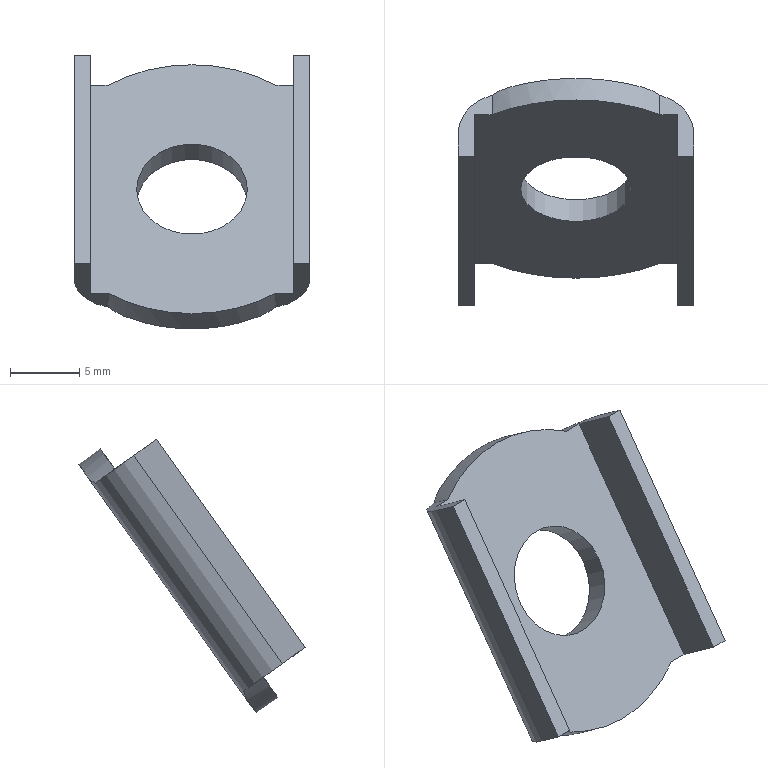Component | SolidWorks | AD12-MC01H-4_2_03.SDASM-1_AD12-_MC01H-4_w.sdprt-2 | 1 solid | 18 faces | box 17.04 x 16.37 x 19.77 mm | volume 623 mm3 | plane 12 | cylinder 6 | commonest cylinder face diameters 8 x2 22.08 x2 7.2 x2
STEP:
#1=COLOUR_RGB('',0.7922,0.8196,0.9333);
#2=FILL_AREA_STYLE_COLOUR('',#1);
#3=FILL_AREA_STYLE('',(#2));
#4=SURFACE_STYLE_FILL_AREA(#3);
#5=SURFACE_SIDE_STYLE('',(#4));
#6=SURFACE_STYLE_USAGE(.BOTH.,#5);
#7=PRESENTATION_STYLE_ASSIGNMENT((#6));
#8=CARTESIAN_POINT('',(-12.123,-7.55,15.022));
#9=VERTEX_POINT('',#8);
#10=CARTESIAN_POINT('',(-12.438,-7.55,15.022));
#11=VERTEX_POINT('',#10);
#12=CARTESIAN_POINT('',(-12.28,-7.55,15.022));
#13=DIRECTION('',(0.,-0.8137,0.5813));
#14=DIRECTION('',(-1.,0.,0.));
#15=AXIS2_PLACEMENT_3D('',#12,#13,#14);
#16=CIRCLE('',#15,0.1575);
#17=EDGE_CURVE('',#9,#11,#16,.T.);
#18=ORIENTED_EDGE('',*,*,#17,.F.);
#19=CARTESIAN_POINT('',(-12.123,-7.611,15.066));
#20=VERTEX_POINT('',#19);
#21=CARTESIAN_POINT('',(-12.123,-7.55,15.022));
#22=DIRECTION('',(0.,-0.8137,0.5813));
#23=VECTOR('',#22,39.37);
#24=LINE('',#21,#23);
#25=EDGE_CURVE('',#9,#20,#24,.T.);
#26=ORIENTED_EDGE('',*,*,#25,.T.);
#27=CARTESIAN_POINT('',(-12.438,-7.611,15.066));
#28=VERTEX_POINT('',#27);
#29=CARTESIAN_POINT('',(-12.28,-7.611,15.066));
#30=DIRECTION('',(0.,-0.8137,0.5813));
#31=DIRECTION('',(-1.,0.,0.));
#32=AXIS2_PLACEMENT_3D('',#29,#30,#31);
#33=CIRCLE('',#32,0.1575);
#34=EDGE_CURVE('',#20,#28,#33,.T.);
#35=ORIENTED_EDGE('',*,*,#34,.T.);
#36=CARTESIAN_POINT('',(-12.438,-7.55,15.022));
#37=DIRECTION('',(0.,-0.8137,0.5813));
#38=VECTOR('',#37,39.37);
#39=LINE('',#36,#38);
#40=EDGE_CURVE('',#11,#28,#39,.T.);
#41=ORIENTED_EDGE('',*,*,#40,.F.);
#42=EDGE_LOOP('',(#18,#26,#35,#41));
#43=FACE_OUTER_BOUND('',#42,.T.);
#44=CARTESIAN_POINT('',(-12.28,-7.55,15.022));
#45=DIRECTION('',(0.,-0.8137,0.5813));
#46=DIRECTION('',(-1.,0.,0.));
#47=AXIS2_PLACEMENT_3D('',#44,#45,#46);
#48=CYLINDRICAL_SURFACE('',#47,0.1575);
#49=ADVANCED_FACE('',(#43),#48,.F.);
#50=CARTESIAN_POINT('',(-12.28,-7.611,15.066));
#51=DIRECTION('',(0.,-0.8137,0.5813));
#52=DIRECTION('',(-1.,0.,0.));
#53=AXIS2_PLACEMENT_3D('',#50,#51,#52);
#54=CIRCLE('',#53,0.1575);
#55=EDGE_CURVE('',#28,#20,#54,.T.);
#56=ORIENTED_EDGE('',*,*,#55,.F.);
#57=ORIENTED_EDGE('',*,*,#34,.F.);
#58=EDGE_LOOP('',(#56,#57));
#59=FACE_BOUND('',#58,.T.);
#60=CARTESIAN_POINT('',(-12.042,-7.823,14.77));
#61=VERTEX_POINT('',#60);
#62=CARTESIAN_POINT('',(-11.991,-7.823,14.77));
#63=VERTEX_POINT('',#62);
#64=CARTESIAN_POINT('',(-12.042,-7.823,14.77));
#65=DIRECTION('',(1.,0.,0.));
#66=VECTOR('',#65,39.37);
#67=LINE('',#64,#66);
#68=EDGE_CURVE('',#61,#63,#67,.T.);
#69=ORIENTED_EDGE('',*,*,#68,.T.);
#70=CARTESIAN_POINT('',(-11.991,-7.4,15.361));
#71=VERTEX_POINT('',#70);
#72=CARTESIAN_POINT('',(-11.991,-7.955,14.585));
#73=DIRECTION('',(0.,-0.5813,-0.8137));
#74=VECTOR('',#73,39.37);
#75=LINE('',#72,#74);
#76=EDGE_CURVE('',#71,#63,#75,.T.);
#77=ORIENTED_EDGE('',*,*,#76,.F.);
#78=CARTESIAN_POINT('',(-12.042,-7.4,15.361));
#79=VERTEX_POINT('',#78);
#80=CARTESIAN_POINT('',(-11.945,-7.4,15.361));
#81=DIRECTION('',(-1.,-0.,0.));
#82=VECTOR('',#81,39.37);
#83=LINE('',#80,#82);
#84=EDGE_CURVE('',#71,#79,#83,.T.);
#85=ORIENTED_EDGE('',*,*,#84,.T.);
#86=CARTESIAN_POINT('',(-12.519,-7.4,15.361));
#87=VERTEX_POINT('',#86);
#88=CARTESIAN_POINT('',(-12.28,-7.611,15.066));
#89=DIRECTION('',(-0.,0.8137,-0.5813));
#90=DIRECTION('',(-1.,-0.,0.));
#91=AXIS2_PLACEMENT_3D('',#88,#89,#90);
#92=CIRCLE('',#91,0.4346);
#93=EDGE_CURVE('',#87,#79,#92,.T.);
#94=ORIENTED_EDGE('',*,*,#93,.F.);
#95=CARTESIAN_POINT('',(-12.569,-7.4,15.361));
#96=VERTEX_POINT('',#95);
#97=CARTESIAN_POINT('',(-12.519,-7.4,15.361));
#98=DIRECTION('',(-1.,-0.,-0.));
#99=VECTOR('',#98,39.37);
#100=LINE('',#97,#99);
#101=EDGE_CURVE('',#87,#96,#100,.T.);
#102=ORIENTED_EDGE('',*,*,#101,.T.);
#103=CARTESIAN_POINT('',(-12.569,-7.823,14.77));
#104=VERTEX_POINT('',#103);
#105=CARTESIAN_POINT('',(-12.569,-7.955,14.585));
#106=DIRECTION('',(-0.,0.5813,0.8137));
#107=VECTOR('',#106,39.37);
#108=LINE('',#105,#107);
#109=EDGE_CURVE('',#104,#96,#108,.T.);
#110=ORIENTED_EDGE('',*,*,#109,.F.);
#111=CARTESIAN_POINT('',(-12.519,-7.823,14.77));
#112=VERTEX_POINT('',#111);
#113=CARTESIAN_POINT('',(-12.616,-7.823,14.77));
#114=DIRECTION('',(1.,0.,0.));
#115=VECTOR('',#114,39.37);
#116=LINE('',#113,#115);
#117=EDGE_CURVE('',#104,#112,#116,.T.);
#118=ORIENTED_EDGE('',*,*,#117,.T.);
#119=CARTESIAN_POINT('',(-12.28,-7.611,15.066));
#120=DIRECTION('',(-0.,0.8137,-0.5813));
#121=DIRECTION('',(-1.,-0.,-0.));
#122=AXIS2_PLACEMENT_3D('',#119,#120,#121);
#123=CIRCLE('',#122,0.4346);
#124=EDGE_CURVE('',#61,#112,#123,.T.);
#125=ORIENTED_EDGE('',*,*,#124,.F.);
#126=EDGE_LOOP('',(#69,#77,#85,#94,#102,#110,#118,#125));
#127=FACE_OUTER_BOUND('',#126,.T.);
#128=CARTESIAN_POINT('',(-11.991,-7.955,14.585));
#129=DIRECTION('',(-0.,0.8137,-0.5813));
#130=DIRECTION('',(1.,0.,0.));
#131=AXIS2_PLACEMENT_3D('',#128,#129,#130);
#132=PLANE('',#131);
#133=ADVANCED_FACE('',(#59,#127),#132,.F.);
#134=ORIENTED_EDGE('',*,*,#25,.F.);
#135=CARTESIAN_POINT('',(-12.28,-7.55,15.022));
#136=DIRECTION('',(0.,-0.8137,0.5813));
#137=DIRECTION('',(-1.,0.,0.));
#138=AXIS2_PLACEMENT_3D('',#135,#136,#137);
#139=CIRCLE('',#138,0.1575);
#140=EDGE_CURVE('',#11,#9,#139,.T.);
#141=ORIENTED_EDGE('',*,*,#140,.F.);
#142=ORIENTED_EDGE('',*,*,#40,.T.);
#143=ORIENTED_EDGE('',*,*,#55,.T.);
#144=EDGE_LOOP('',(#134,#141,#142,#143));
#145=FACE_OUTER_BOUND('',#144,.T.);
#146=CARTESIAN_POINT('',(-12.28,-7.55,15.022));
#147=DIRECTION('',(0.,-0.8137,0.5813));
#148=DIRECTION('',(-1.,0.,0.));
#149=AXIS2_PLACEMENT_3D('',#146,#147,#148);
#150=CYLINDRICAL_SURFACE('',#149,0.1575);
#151=ADVANCED_FACE('',(#145),#150,.F.);
#152=CARTESIAN_POINT('',(-12.042,-7.767,14.73));
#153=VERTEX_POINT('',#152);
#154=CARTESIAN_POINT('',(-12.042,-8.081,14.955));
#155=DIRECTION('',(0.,-0.8137,0.5813));
#156=VECTOR('',#155,39.37);
#157=LINE('',#154,#156);
#158=EDGE_CURVE('',#153,#61,#157,.T.);
#159=ORIENTED_EDGE('',*,*,#158,.T.);
#160=ORIENTED_EDGE('',*,*,#124,.T.);
#161=CARTESIAN_POINT('',(-12.519,-7.767,14.73));
#162=VERTEX_POINT('',#161);
#163=CARTESIAN_POINT('',(-12.519,-8.081,14.955));
#164=DIRECTION('',(-0.,0.8137,-0.5813));
#165=VECTOR('',#164,39.37);
#166=LINE('',#163,#165);
#167=EDGE_CURVE('',#112,#162,#166,.T.);
#168=ORIENTED_EDGE('',*,*,#167,.T.);
#169=CARTESIAN_POINT('',(-12.474,-7.776,14.705));
#170=VERTEX_POINT('',#169);
#171=CARTESIAN_POINT('',(-12.474,-7.776,14.705));
#172=CARTESIAN_POINT('',(-12.49,-7.771,14.712));
#173=CARTESIAN_POINT('',(-12.504,-7.769,14.72));
#174=CARTESIAN_POINT('',(-12.519,-7.767,14.73));
#175=B_SPLINE_CURVE_WITH_KNOTS('',3,(#171,#172,#173,#174),.UNSPECIFIED.,.F.,.F.,(4,4),(0.,0.001324),.UNSPECIFIED.);
#176=EDGE_CURVE('',#170,#162,#175,.T.);
#177=ORIENTED_EDGE('',*,*,#176,.F.);
#178=CARTESIAN_POINT('',(-12.086,-7.776,14.705));
#179=VERTEX_POINT('',#178);
#180=CARTESIAN_POINT('',(-12.28,-7.55,15.022));
#181=DIRECTION('',(0.,-0.8137,0.5813));
#182=DIRECTION('',(-1.,0.,0.));
#183=AXIS2_PLACEMENT_3D('',#180,#181,#182);
#184=CIRCLE('',#183,0.4346);
#185=EDGE_CURVE('',#170,#179,#184,.T.);
#186=ORIENTED_EDGE('',*,*,#185,.T.);
#187=CARTESIAN_POINT('',(-12.042,-7.767,14.73));
#188=CARTESIAN_POINT('',(-12.056,-7.769,14.72));
#189=CARTESIAN_POINT('',(-12.071,-7.771,14.712));
#190=CARTESIAN_POINT('',(-12.086,-7.776,14.705));
#191=B_SPLINE_CURVE_WITH_KNOTS('',3,(#187,#188,#189,#190),.UNSPECIFIED.,.F.,.F.,(4,4),(0.,0.001324),.UNSPECIFIED.);
#192=EDGE_CURVE('',#153,#179,#191,.T.);
#193=ORIENTED_EDGE('',*,*,#192,.F.);
#194=EDGE_LOOP('',(#159,#160,#168,#177,#186,#193));
#195=FACE_OUTER_BOUND('',#194,.T.);
#196=CARTESIAN_POINT('',(-12.28,-7.87,15.251));
#197=DIRECTION('',(0.,-0.8137,0.5813));
#198=DIRECTION('',(-1.,0.,0.));
#199=AXIS2_PLACEMENT_3D('',#196,#197,#198);
#200=CYLINDRICAL_SURFACE('',#199,0.4346);
#201=ADVANCED_FACE('',(#195),#200,.T.);
#202=CARTESIAN_POINT('',(-11.991,-7.519,15.447));
#203=VERTEX_POINT('',#202);
#204=CARTESIAN_POINT('',(-11.991,-7.519,15.447));
#205=DIRECTION('',(0.,-0.8137,0.5813));
#206=VECTOR('',#205,39.37);
#207=LINE('',#204,#206);
#208=EDGE_CURVE('',#71,#203,#207,.T.);
#209=ORIENTED_EDGE('',*,*,#208,.F.);
#210=ORIENTED_EDGE('',*,*,#76,.T.);
#211=CARTESIAN_POINT('',(-11.991,-7.942,14.855));
#212=VERTEX_POINT('',#211);
#213=CARTESIAN_POINT('',(-11.991,-7.942,14.855));
#214=DIRECTION('',(-0.,0.8137,-0.5813));
#215=VECTOR('',#214,39.37);
#216=LINE('',#213,#215);
#217=EDGE_CURVE('',#212,#63,#216,.T.);
#218=ORIENTED_EDGE('',*,*,#217,.F.);
#219=CARTESIAN_POINT('',(-11.991,-8.074,14.67));
#220=DIRECTION('',(0.,-0.5813,-0.8137));
#221=VECTOR('',#220,39.37);
#222=LINE('',#219,#221);
#223=EDGE_CURVE('',#203,#212,#222,.T.);
#224=ORIENTED_EDGE('',*,*,#223,.F.);
#225=EDGE_LOOP('',(#209,#210,#218,#224));
#226=FACE_OUTER_BOUND('',#225,.T.);
#227=CARTESIAN_POINT('',(-11.991,-8.074,14.67));
#228=DIRECTION('',(1.,0.,0.));
#229=DIRECTION('',(-0.,0.5813,0.8137));
#230=AXIS2_PLACEMENT_3D('',#227,#228,#229);
#231=PLANE('',#230);
#232=ADVANCED_FACE('',(#226),#231,.F.);
#233=CARTESIAN_POINT('',(-12.519,-7.345,15.322));
#234=VERTEX_POINT('',#233);
#235=CARTESIAN_POINT('',(-12.519,-7.659,15.546));
#236=DIRECTION('',(0.,-0.8137,0.5813));
#237=VECTOR('',#236,39.37);
#238=LINE('',#235,#237);
#239=EDGE_CURVE('',#234,#87,#238,.T.);
#240=ORIENTED_EDGE('',*,*,#239,.T.);
#241=ORIENTED_EDGE('',*,*,#93,.T.);
#242=CARTESIAN_POINT('',(-12.042,-7.345,15.322));
#243=VERTEX_POINT('',#242);
#244=CARTESIAN_POINT('',(-12.042,-7.659,15.546));
#245=DIRECTION('',(-0.,0.8137,-0.5813));
#246=VECTOR('',#245,39.37);
#247=LINE('',#244,#246);
#248=EDGE_CURVE('',#79,#243,#247,.T.);
#249=ORIENTED_EDGE('',*,*,#248,.T.);
#250=CARTESIAN_POINT('',(-12.086,-7.324,15.338));
#251=VERTEX_POINT('',#250);
#252=CARTESIAN_POINT('',(-12.086,-7.324,15.338));
#253=CARTESIAN_POINT('',(-12.071,-7.328,15.332));
#254=CARTESIAN_POINT('',(-12.056,-7.335,15.326));
#255=CARTESIAN_POINT('',(-12.042,-7.345,15.322));
#256=B_SPLINE_CURVE_WITH_KNOTS('',3,(#252,#253,#254,#255),.UNSPECIFIED.,.F.,.F.,(4,4),(0.,0.001324),.UNSPECIFIED.);
#257=EDGE_CURVE('',#251,#243,#256,.T.);
#258=ORIENTED_EDGE('',*,*,#257,.F.);
#259=CARTESIAN_POINT('',(-12.474,-7.324,15.338));
#260=VERTEX_POINT('',#259);
#261=CARTESIAN_POINT('',(-12.28,-7.55,15.022));
#262=DIRECTION('',(0.,-0.8137,0.5813));
#263=DIRECTION('',(-1.,0.,0.));
#264=AXIS2_PLACEMENT_3D('',#261,#262,#263);
#265=CIRCLE('',#264,0.4346);
#266=EDGE_CURVE('',#251,#260,#265,.T.);
#267=ORIENTED_EDGE('',*,*,#266,.T.);
#268=CARTESIAN_POINT('',(-12.519,-7.345,15.322));
#269=CARTESIAN_POINT('',(-12.504,-7.335,15.326));
#270=CARTESIAN_POINT('',(-12.49,-7.328,15.332));
#271=CARTESIAN_POINT('',(-12.474,-7.324,15.338));
#272=B_SPLINE_CURVE_WITH_KNOTS('',3,(#268,#269,#270,#271),.UNSPECIFIED.,.F.,.F.,(4,4),(0.,0.001324),.UNSPECIFIED.);
#273=EDGE_CURVE('',#234,#260,#272,.T.);
#274=ORIENTED_EDGE('',*,*,#273,.F.);
#275=EDGE_LOOP('',(#240,#241,#249,#258,#267,#274));
#276=FACE_OUTER_BOUND('',#275,.T.);
#277=CARTESIAN_POINT('',(-12.28,-7.87,15.251));
#278=DIRECTION('',(0.,-0.8137,0.5813));
#279=DIRECTION('',(-1.,0.,0.));
#280=AXIS2_PLACEMENT_3D('',#277,#278,#279);
#281=CYLINDRICAL_SURFACE('',#280,0.4346);
#282=ADVANCED_FACE('',(#276),#281,.T.);
#283=CARTESIAN_POINT('',(-12.569,-7.942,14.855));
#284=VERTEX_POINT('',#283);
#285=CARTESIAN_POINT('',(-12.569,-7.823,14.77));
#286=DIRECTION('',(0.,-0.8137,0.5813));
#287=VECTOR('',#286,39.37);
#288=LINE('',#285,#287);
#289=EDGE_CURVE('',#104,#284,#288,.T.);
#290=ORIENTED_EDGE('',*,*,#289,.F.);
#291=ORIENTED_EDGE('',*,*,#109,.T.);
#292=CARTESIAN_POINT('',(-12.569,-7.519,15.447));
#293=VERTEX_POINT('',#292);
#294=CARTESIAN_POINT('',(-12.569,-7.4,15.361));
#295=DIRECTION('',(-0.,0.8137,-0.5813));
#296=VECTOR('',#295,39.37);
#297=LINE('',#294,#296);
#298=EDGE_CURVE('',#293,#96,#297,.T.);
#299=ORIENTED_EDGE('',*,*,#298,.F.);
#300=CARTESIAN_POINT('',(-12.569,-8.074,14.67));
#301=DIRECTION('',(-0.,0.5813,0.8137));
#302=VECTOR('',#301,39.37);
#303=LINE('',#300,#302);
#304=EDGE_CURVE('',#284,#293,#303,.T.);
#305=ORIENTED_EDGE('',*,*,#304,.F.);
#306=EDGE_LOOP('',(#290,#291,#299,#305));
#307=FACE_OUTER_BOUND('',#306,.T.);
#308=CARTESIAN_POINT('',(-12.569,-7.955,14.585));
#309=DIRECTION('',(-1.,-0.,-0.));
#310=DIRECTION('',(0.,-0.5813,-0.8137));
#311=AXIS2_PLACEMENT_3D('',#308,#309,#310);
#312=PLANE('',#311);
#313=ADVANCED_FACE('',(#307),#312,.F.);
#314=ORIENTED_EDGE('',*,*,#140,.T.);
#315=ORIENTED_EDGE('',*,*,#17,.T.);
#316=EDGE_LOOP('',(#314,#315));
#317=FACE_BOUND('',#316,.T.);
#318=ORIENTED_EDGE('',*,*,#185,.F.);
#319=CARTESIAN_POINT('',(-12.474,-7.893,14.541));
#320=DIRECTION('',(0.,-0.5813,-0.8137));
#321=VECTOR('',#320,39.37);
#322=LINE('',#319,#321);
#323=EDGE_CURVE('',#260,#170,#322,.T.);
#324=ORIENTED_EDGE('',*,*,#323,.F.);
#325=ORIENTED_EDGE('',*,*,#266,.F.);
#326=CARTESIAN_POINT('',(-12.086,-7.893,14.541));
#327=DIRECTION('',(-0.,0.5813,0.8137));
#328=VECTOR('',#327,39.37);
#329=LINE('',#326,#328);
#330=EDGE_CURVE('',#179,#251,#329,.T.);
#331=ORIENTED_EDGE('',*,*,#330,.F.);
#332=EDGE_LOOP('',(#318,#324,#325,#331));
#333=FACE_OUTER_BOUND('',#332,.T.);
#334=CARTESIAN_POINT('',(-12.674,-7.893,14.541));
#335=DIRECTION('',(0.,-0.8137,0.5813));
#336=DIRECTION('',(-1.,-0.,-0.));
#337=AXIS2_PLACEMENT_3D('',#334,#335,#336);
#338=PLANE('',#337);
#339=ADVANCED_FACE('',(#317,#333),#338,.F.);
#340=CARTESIAN_POINT('',(-11.945,-7.876,14.808));
#341=VERTEX_POINT('',#340);
#342=CARTESIAN_POINT('',(-12.086,-7.876,14.808));
#343=DIRECTION('',(-0.,0.5813,0.8137));
#344=DIRECTION('',(1.,0.,0.));
#345=AXIS2_PLACEMENT_3D('',#342,#343,#344);
#346=CIRCLE('',#345,0.1417);
#347=EDGE_CURVE('',#341,#153,#346,.T.);
#348=ORIENTED_EDGE('',*,*,#347,.F.);
#349=CARTESIAN_POINT('',(-11.945,-7.942,14.855));
#350=VERTEX_POINT('',#349);
#351=CARTESIAN_POINT('',(-11.945,-8.081,14.955));
#352=DIRECTION('',(-0.,0.8137,-0.5813));
#353=VECTOR('',#352,39.37);
#354=LINE('',#351,#353);
#355=EDGE_CURVE('',#350,#341,#354,.T.);
#356=ORIENTED_EDGE('',*,*,#355,.F.);
#357=CARTESIAN_POINT('',(-12.042,-7.942,14.855));
#358=DIRECTION('',(1.,0.,0.));
#359=VECTOR('',#358,39.37);
#360=LINE('',#357,#359);
#361=EDGE_CURVE('',#212,#350,#360,.T.);
#362=ORIENTED_EDGE('',*,*,#361,.F.);
#363=ORIENTED_EDGE('',*,*,#217,.T.);
#364=ORIENTED_EDGE('',*,*,#68,.F.);
#365=ORIENTED_EDGE('',*,*,#158,.F.);
#366=EDGE_LOOP('',(#348,#356,#362,#363,#364,#365));
#367=FACE_OUTER_BOUND('',#366,.T.);
#368=CARTESIAN_POINT('',(-12.042,-8.081,14.955));
#369=DIRECTION('',(-0.,0.5813,0.8137));
#370=DIRECTION('',(-1.,-0.,-0.));
#371=AXIS2_PLACEMENT_3D('',#368,#369,#370);
#372=PLANE('',#371);
#373=ADVANCED_FACE('',(#367),#372,.F.);
#374=CARTESIAN_POINT('',(-12.616,-7.876,14.808));
#375=VERTEX_POINT('',#374);
#376=CARTESIAN_POINT('',(-12.474,-7.876,14.808));
#377=DIRECTION('',(-0.,0.5813,0.8137));
#378=DIRECTION('',(1.,0.,0.));
#379=AXIS2_PLACEMENT_3D('',#376,#377,#378);
#380=CIRCLE('',#379,0.1417);
#381=EDGE_CURVE('',#162,#375,#380,.T.);
#382=ORIENTED_EDGE('',*,*,#381,.F.);
#383=ORIENTED_EDGE('',*,*,#167,.F.);
#384=ORIENTED_EDGE('',*,*,#117,.F.);
#385=ORIENTED_EDGE('',*,*,#289,.T.);
#386=CARTESIAN_POINT('',(-12.616,-7.942,14.855));
#387=VERTEX_POINT('',#386);
#388=CARTESIAN_POINT('',(-12.616,-7.942,14.855));
#389=DIRECTION('',(1.,0.,0.));
#390=VECTOR('',#389,39.37);
#391=LINE('',#388,#390);
#392=EDGE_CURVE('',#387,#284,#391,.T.);
#393=ORIENTED_EDGE('',*,*,#392,.F.);
#394=CARTESIAN_POINT('',(-12.616,-8.081,14.955));
#395=DIRECTION('',(0.,-0.8137,0.5813));
#396=VECTOR('',#395,39.37);
#397=LINE('',#394,#396);
#398=EDGE_CURVE('',#375,#387,#397,.T.);
#399=ORIENTED_EDGE('',*,*,#398,.F.);
#400=EDGE_LOOP('',(#382,#383,#384,#385,#393,#399));
#401=FACE_OUTER_BOUND('',#400,.T.);
#402=CARTESIAN_POINT('',(-12.616,-8.081,14.955));
#403=DIRECTION('',(-0.,0.5813,0.8137));
#404=DIRECTION('',(-1.,-0.,-0.));
#405=AXIS2_PLACEMENT_3D('',#402,#403,#404);
#406=PLANE('',#405);
#407=ADVANCED_FACE('',(#401),#406,.F.);
#408=CARTESIAN_POINT('',(-11.945,-7.519,15.447));
#409=VERTEX_POINT('',#408);
#410=CARTESIAN_POINT('',(-11.945,-7.519,15.447));
#411=DIRECTION('',(1.,0.,0.));
#412=VECTOR('',#411,39.37);
#413=LINE('',#410,#412);
#414=EDGE_CURVE('',#203,#409,#413,.T.);
#415=ORIENTED_EDGE('',*,*,#414,.F.);
#416=ORIENTED_EDGE('',*,*,#223,.T.);
#417=ORIENTED_EDGE('',*,*,#361,.T.);
#418=CARTESIAN_POINT('',(-11.945,-8.074,14.67));
#419=DIRECTION('',(0.,-0.5813,-0.8137));
#420=VECTOR('',#419,39.37);
#421=LINE('',#418,#420);
#422=EDGE_CURVE('',#409,#350,#421,.T.);
#423=ORIENTED_EDGE('',*,*,#422,.F.);
#424=EDGE_LOOP('',(#415,#416,#417,#423));
#425=FACE_OUTER_BOUND('',#424,.T.);
#426=CARTESIAN_POINT('',(-11.945,-8.074,14.67));
#427=DIRECTION('',(-0.,0.8137,-0.5813));
#428=DIRECTION('',(1.,0.,0.));
#429=AXIS2_PLACEMENT_3D('',#426,#427,#428);
#430=PLANE('',#429);
#431=ADVANCED_FACE('',(#425),#430,.F.);
#432=ORIENTED_EDGE('',*,*,#414,.T.);
#433=CARTESIAN_POINT('',(-11.945,-7.454,15.4));
#434=VERTEX_POINT('',#433);
#435=CARTESIAN_POINT('',(-11.945,-7.659,15.546));
#436=DIRECTION('',(0.,-0.8137,0.5813));
#437=VECTOR('',#436,39.37);
#438=LINE('',#435,#437);
#439=EDGE_CURVE('',#434,#409,#438,.T.);
#440=ORIENTED_EDGE('',*,*,#439,.F.);
#441=CARTESIAN_POINT('',(-12.086,-7.454,15.4));
#442=DIRECTION('',(0.,-0.5813,-0.8137));
#443=DIRECTION('',(1.,0.,0.));
#444=AXIS2_PLACEMENT_3D('',#441,#442,#443);
#445=CIRCLE('',#444,0.1417);
#446=EDGE_CURVE('',#243,#434,#445,.T.);
#447=ORIENTED_EDGE('',*,*,#446,.F.);
#448=ORIENTED_EDGE('',*,*,#248,.F.);
#449=ORIENTED_EDGE('',*,*,#84,.F.);
#450=ORIENTED_EDGE('',*,*,#208,.T.);
#451=EDGE_LOOP('',(#432,#440,#447,#448,#449,#450));
#452=FACE_OUTER_BOUND('',#451,.T.);
#453=CARTESIAN_POINT('',(-11.945,-7.659,15.546));
#454=DIRECTION('',(-0.,-0.5813,-0.8137));
#455=DIRECTION('',(1.,0.,-0.));
#456=AXIS2_PLACEMENT_3D('',#453,#454,#455);
#457=PLANE('',#456);
#458=ADVANCED_FACE('',(#452),#457,.F.);
#459=ORIENTED_EDGE('',*,*,#101,.F.);
#460=ORIENTED_EDGE('',*,*,#239,.F.);
#461=CARTESIAN_POINT('',(-12.616,-7.454,15.4));
#462=VERTEX_POINT('',#461);
#463=CARTESIAN_POINT('',(-12.474,-7.454,15.4));
#464=DIRECTION('',(0.,-0.5813,-0.8137));
#465=DIRECTION('',(1.,0.,0.));
#466=AXIS2_PLACEMENT_3D('',#463,#464,#465);
#467=CIRCLE('',#466,0.1417);
#468=EDGE_CURVE('',#462,#234,#467,.T.);
#469=ORIENTED_EDGE('',*,*,#468,.F.);
#470=CARTESIAN_POINT('',(-12.616,-7.519,15.447));
#471=VERTEX_POINT('',#470);
#472=CARTESIAN_POINT('',(-12.616,-7.659,15.546));
#473=DIRECTION('',(-0.,0.8137,-0.5813));
#474=VECTOR('',#473,39.37);
#475=LINE('',#472,#474);
#476=EDGE_CURVE('',#471,#462,#475,.T.);
#477=ORIENTED_EDGE('',*,*,#476,.F.);
#478=CARTESIAN_POINT('',(-12.519,-7.519,15.447));
#479=DIRECTION('',(-1.,-0.,-0.));
#480=VECTOR('',#479,39.37);
#481=LINE('',#478,#480);
#482=EDGE_CURVE('',#293,#471,#481,.T.);
#483=ORIENTED_EDGE('',*,*,#482,.F.);
#484=ORIENTED_EDGE('',*,*,#298,.T.);
#485=EDGE_LOOP('',(#459,#460,#469,#477,#483,#484));
#486=FACE_OUTER_BOUND('',#485,.T.);
#487=CARTESIAN_POINT('',(-12.519,-7.659,15.546));
#488=DIRECTION('',(0.,-0.5813,-0.8137));
#489=DIRECTION('',(1.,0.,0.));
#490=AXIS2_PLACEMENT_3D('',#487,#488,#489);
#491=PLANE('',#490);
#492=ADVANCED_FACE('',(#486),#491,.F.);
#493=ORIENTED_EDGE('',*,*,#392,.T.);
#494=ORIENTED_EDGE('',*,*,#304,.T.);
#495=ORIENTED_EDGE('',*,*,#482,.T.);
#496=CARTESIAN_POINT('',(-12.616,-8.074,14.67));
#497=DIRECTION('',(-0.,0.5813,0.8137));
#498=VECTOR('',#497,39.37);
#499=LINE('',#496,#498);
#500=EDGE_CURVE('',#387,#471,#499,.T.);
#501=ORIENTED_EDGE('',*,*,#500,.F.);
#502=EDGE_LOOP('',(#493,#494,#495,#501));
#503=FACE_OUTER_BOUND('',#502,.T.);
#504=CARTESIAN_POINT('',(-12.569,-8.074,14.67));
#505=DIRECTION('',(0.,0.8137,-0.5813));
#506=DIRECTION('',(1.,0.,0.));
#507=AXIS2_PLACEMENT_3D('',#504,#505,#506);
#508=PLANE('',#507);
#509=ADVANCED_FACE('',(#503),#508,.F.);
#510=ORIENTED_EDGE('',*,*,#257,.T.);
#511=ORIENTED_EDGE('',*,*,#446,.T.);
#512=CARTESIAN_POINT('',(-11.945,-8.008,14.624));
#513=DIRECTION('',(0.,-0.5813,-0.8137));
#514=VECTOR('',#513,39.37);
#515=LINE('',#512,#514);
#516=EDGE_CURVE('',#434,#341,#515,.T.);
#517=ORIENTED_EDGE('',*,*,#516,.T.);
#518=ORIENTED_EDGE('',*,*,#347,.T.);
#519=ORIENTED_EDGE('',*,*,#192,.T.);
#520=ORIENTED_EDGE('',*,*,#330,.T.);
#521=EDGE_LOOP('',(#510,#511,#517,#518,#519,#520));
#522=FACE_OUTER_BOUND('',#521,.T.);
#523=CARTESIAN_POINT('',(-12.086,-8.008,14.624));
#524=DIRECTION('',(0.,-0.5813,-0.8137));
#525=DIRECTION('',(1.,0.,0.));
#526=AXIS2_PLACEMENT_3D('',#523,#524,#525);
#527=CYLINDRICAL_SURFACE('',#526,0.1417);
#528=ADVANCED_FACE('',(#522),#527,.T.);
#529=ORIENTED_EDGE('',*,*,#468,.T.);
#530=ORIENTED_EDGE('',*,*,#273,.T.);
#531=ORIENTED_EDGE('',*,*,#323,.T.);
#532=ORIENTED_EDGE('',*,*,#176,.T.);
#533=ORIENTED_EDGE('',*,*,#381,.T.);
#534=CARTESIAN_POINT('',(-12.616,-8.008,14.624));
#535=DIRECTION('',(-0.,0.5813,0.8137));
#536=VECTOR('',#535,39.37);
#537=LINE('',#534,#536);
#538=EDGE_CURVE('',#375,#462,#537,.T.);
#539=ORIENTED_EDGE('',*,*,#538,.T.);
#540=EDGE_LOOP('',(#529,#530,#531,#532,#533,#539));
#541=FACE_OUTER_BOUND('',#540,.T.);
#542=CARTESIAN_POINT('',(-12.474,-8.008,14.624));
#543=DIRECTION('',(0.,-0.5813,-0.8137));
#544=DIRECTION('',(1.,0.,0.));
#545=AXIS2_PLACEMENT_3D('',#542,#543,#544);
#546=CYLINDRICAL_SURFACE('',#545,0.1417);
#547=ADVANCED_FACE('',(#541),#546,.T.);
#548=ORIENTED_EDGE('',*,*,#439,.T.);
#549=ORIENTED_EDGE('',*,*,#422,.T.);
#550=ORIENTED_EDGE('',*,*,#355,.T.);
#551=ORIENTED_EDGE('',*,*,#516,.F.);
#552=EDGE_LOOP('',(#548,#549,#550,#551));
#553=FACE_OUTER_BOUND('',#552,.T.);
#554=CARTESIAN_POINT('',(-11.945,-8.008,14.624));
#555=DIRECTION('',(-1.,0.,-0.));
#556=DIRECTION('',(0.,0.8137,-0.5813));
#557=AXIS2_PLACEMENT_3D('',#554,#555,#556);
#558=PLANE('',#557);
#559=ADVANCED_FACE('',(#553),#558,.F.);
#560=ORIENTED_EDGE('',*,*,#398,.T.);
#561=ORIENTED_EDGE('',*,*,#500,.T.);
#562=ORIENTED_EDGE('',*,*,#476,.T.);
#563=ORIENTED_EDGE('',*,*,#538,.F.);
#564=EDGE_LOOP('',(#560,#561,#562,#563));
#565=FACE_OUTER_BOUND('',#564,.T.);
#566=CARTESIAN_POINT('',(-12.616,-8.074,14.67));
#567=DIRECTION('',(1.,0.,-0.));
#568=DIRECTION('',(0.,-0.8137,0.5813));
#569=AXIS2_PLACEMENT_3D('',#566,#567,#568);
#570=PLANE('',#569);
#571=ADVANCED_FACE('',(#565),#570,.F.);
#572=CLOSED_SHELL('',(#49,#133,#151,#201,#232,#282,#313,#339,#373,#407,#431,#458,#492,#509,#528,#547,#559,#571));
#573=MANIFOLD_SOLID_BREP('',#572);
#574=STYLED_ITEM('',(#7),#573);
#575=(LENGTH_UNIT()NAMED_UNIT(*)SI_UNIT($,.METRE.));
#576=LENGTH_MEASURE_WITH_UNIT(LENGTH_MEASURE(0.0254),#575);
#577=DIMENSIONAL_EXPONENTS(1.,0.,0.,0.,0.,0.,0.);
#578=(CONVERSION_BASED_UNIT('',#576)LENGTH_UNIT()NAMED_UNIT(#577));
#579=UNCERTAINTY_MEASURE_WITH_UNIT(LENGTH_MEASURE(0.00001),#578,'','');
#580=(NAMED_UNIT(*)PLANE_ANGLE_UNIT()SI_UNIT($,.RADIAN.));
#581=(NAMED_UNIT(*)SI_UNIT($,.STERADIAN.)SOLID_ANGLE_UNIT());
#582=(GEOMETRIC_REPRESENTATION_CONTEXT(3)GLOBAL_UNCERTAINTY_ASSIGNED_CONTEXT((#579))GLOBAL_UNIT_ASSIGNED_CONTEXT((#578,#580,#581))REPRESENTATION_CONTEXT('',''));
#583=MECHANICAL_DESIGN_GEOMETRIC_PRESENTATION_REPRESENTATION('',(#574),#582);
#584=PRESENTATION_LAYER_ASSIGNMENT('','',(#574));
#585=CARTESIAN_POINT('',(0.,0.,0.));
#586=DIRECTION('',(0.,0.,1.));
#587=DIRECTION('',(1.,0.,0.));
#588=AXIS2_PLACEMENT_3D('',#585,#586,#587);
#589=(LENGTH_UNIT()NAMED_UNIT(*)SI_UNIT($,.METRE.));
#590=LENGTH_MEASURE_WITH_UNIT(LENGTH_MEASURE(0.0254),#589);
#591=DIMENSIONAL_EXPONENTS(1.,0.,0.,0.,0.,0.,0.);
#592=(CONVERSION_BASED_UNIT('',#590)LENGTH_UNIT()NAMED_UNIT(#591));
#593=UNCERTAINTY_MEASURE_WITH_UNIT(LENGTH_MEASURE(0.00001),#592,'','');
#594=(NAMED_UNIT(*)PLANE_ANGLE_UNIT()SI_UNIT($,.RADIAN.));
#595=(NAMED_UNIT(*)SI_UNIT($,.STERADIAN.)SOLID_ANGLE_UNIT());
#596=(GEOMETRIC_REPRESENTATION_CONTEXT(3)GLOBAL_UNCERTAINTY_ASSIGNED_CONTEXT((#593))GLOBAL_UNIT_ASSIGNED_CONTEXT((#592,#594,#595))REPRESENTATION_CONTEXT('',''));
#597=ADVANCED_BREP_SHAPE_REPRESENTATION('',(#573,#588),#596);